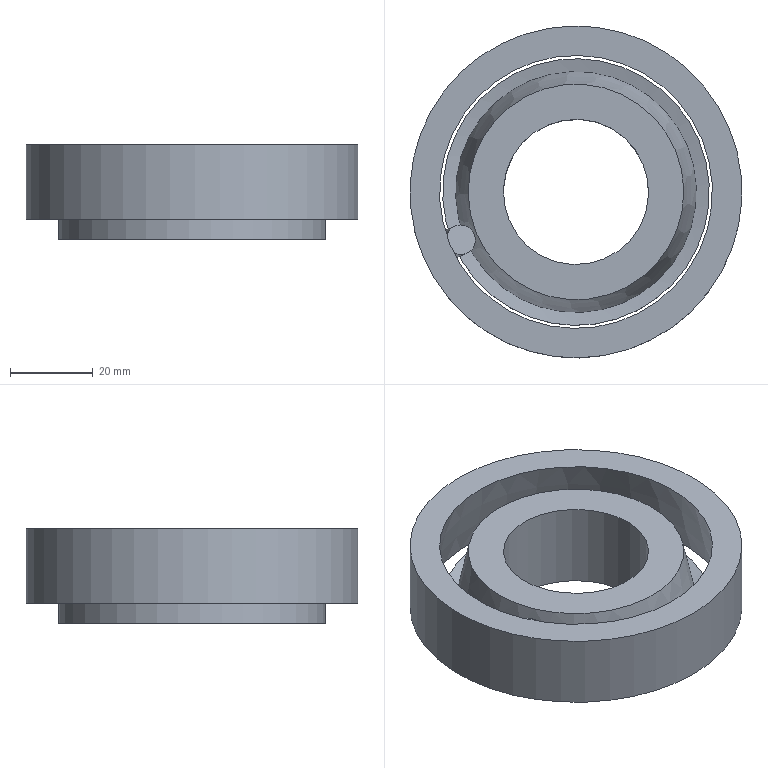Component | NX | CT-ZHOU5-ZHOUCHENG2 | 3 solids | 16 faces | volume 58147 mm3 | plane 6 | cylinder 6 | cone 4 | commonest cylinder face diameters 64.269 x3 35 x1 7.115 x1 80 x1